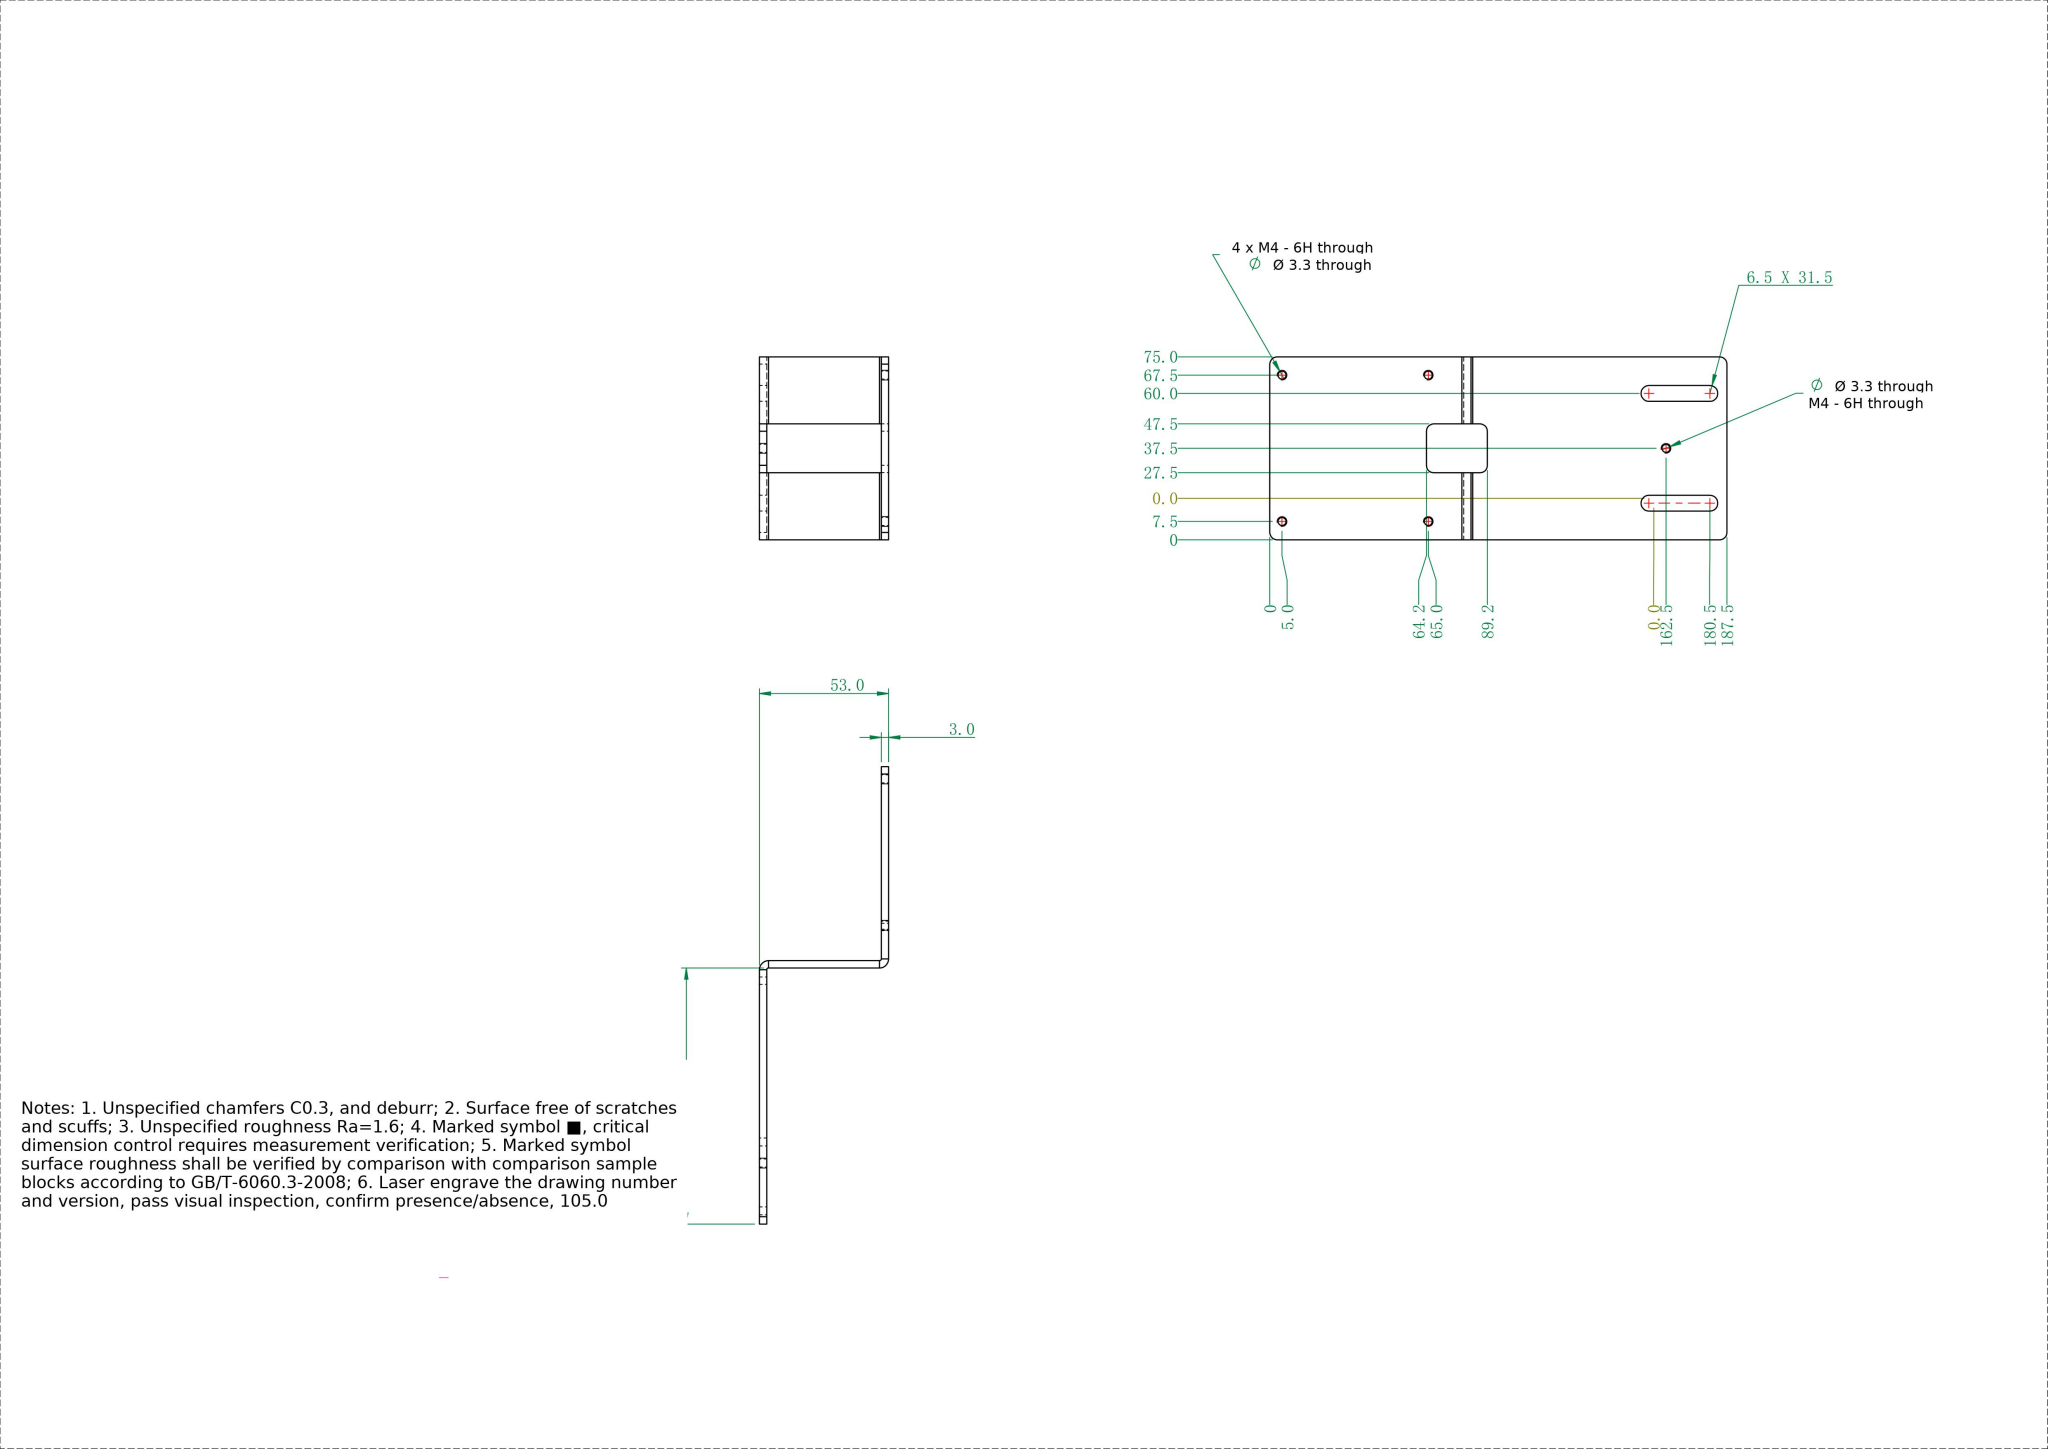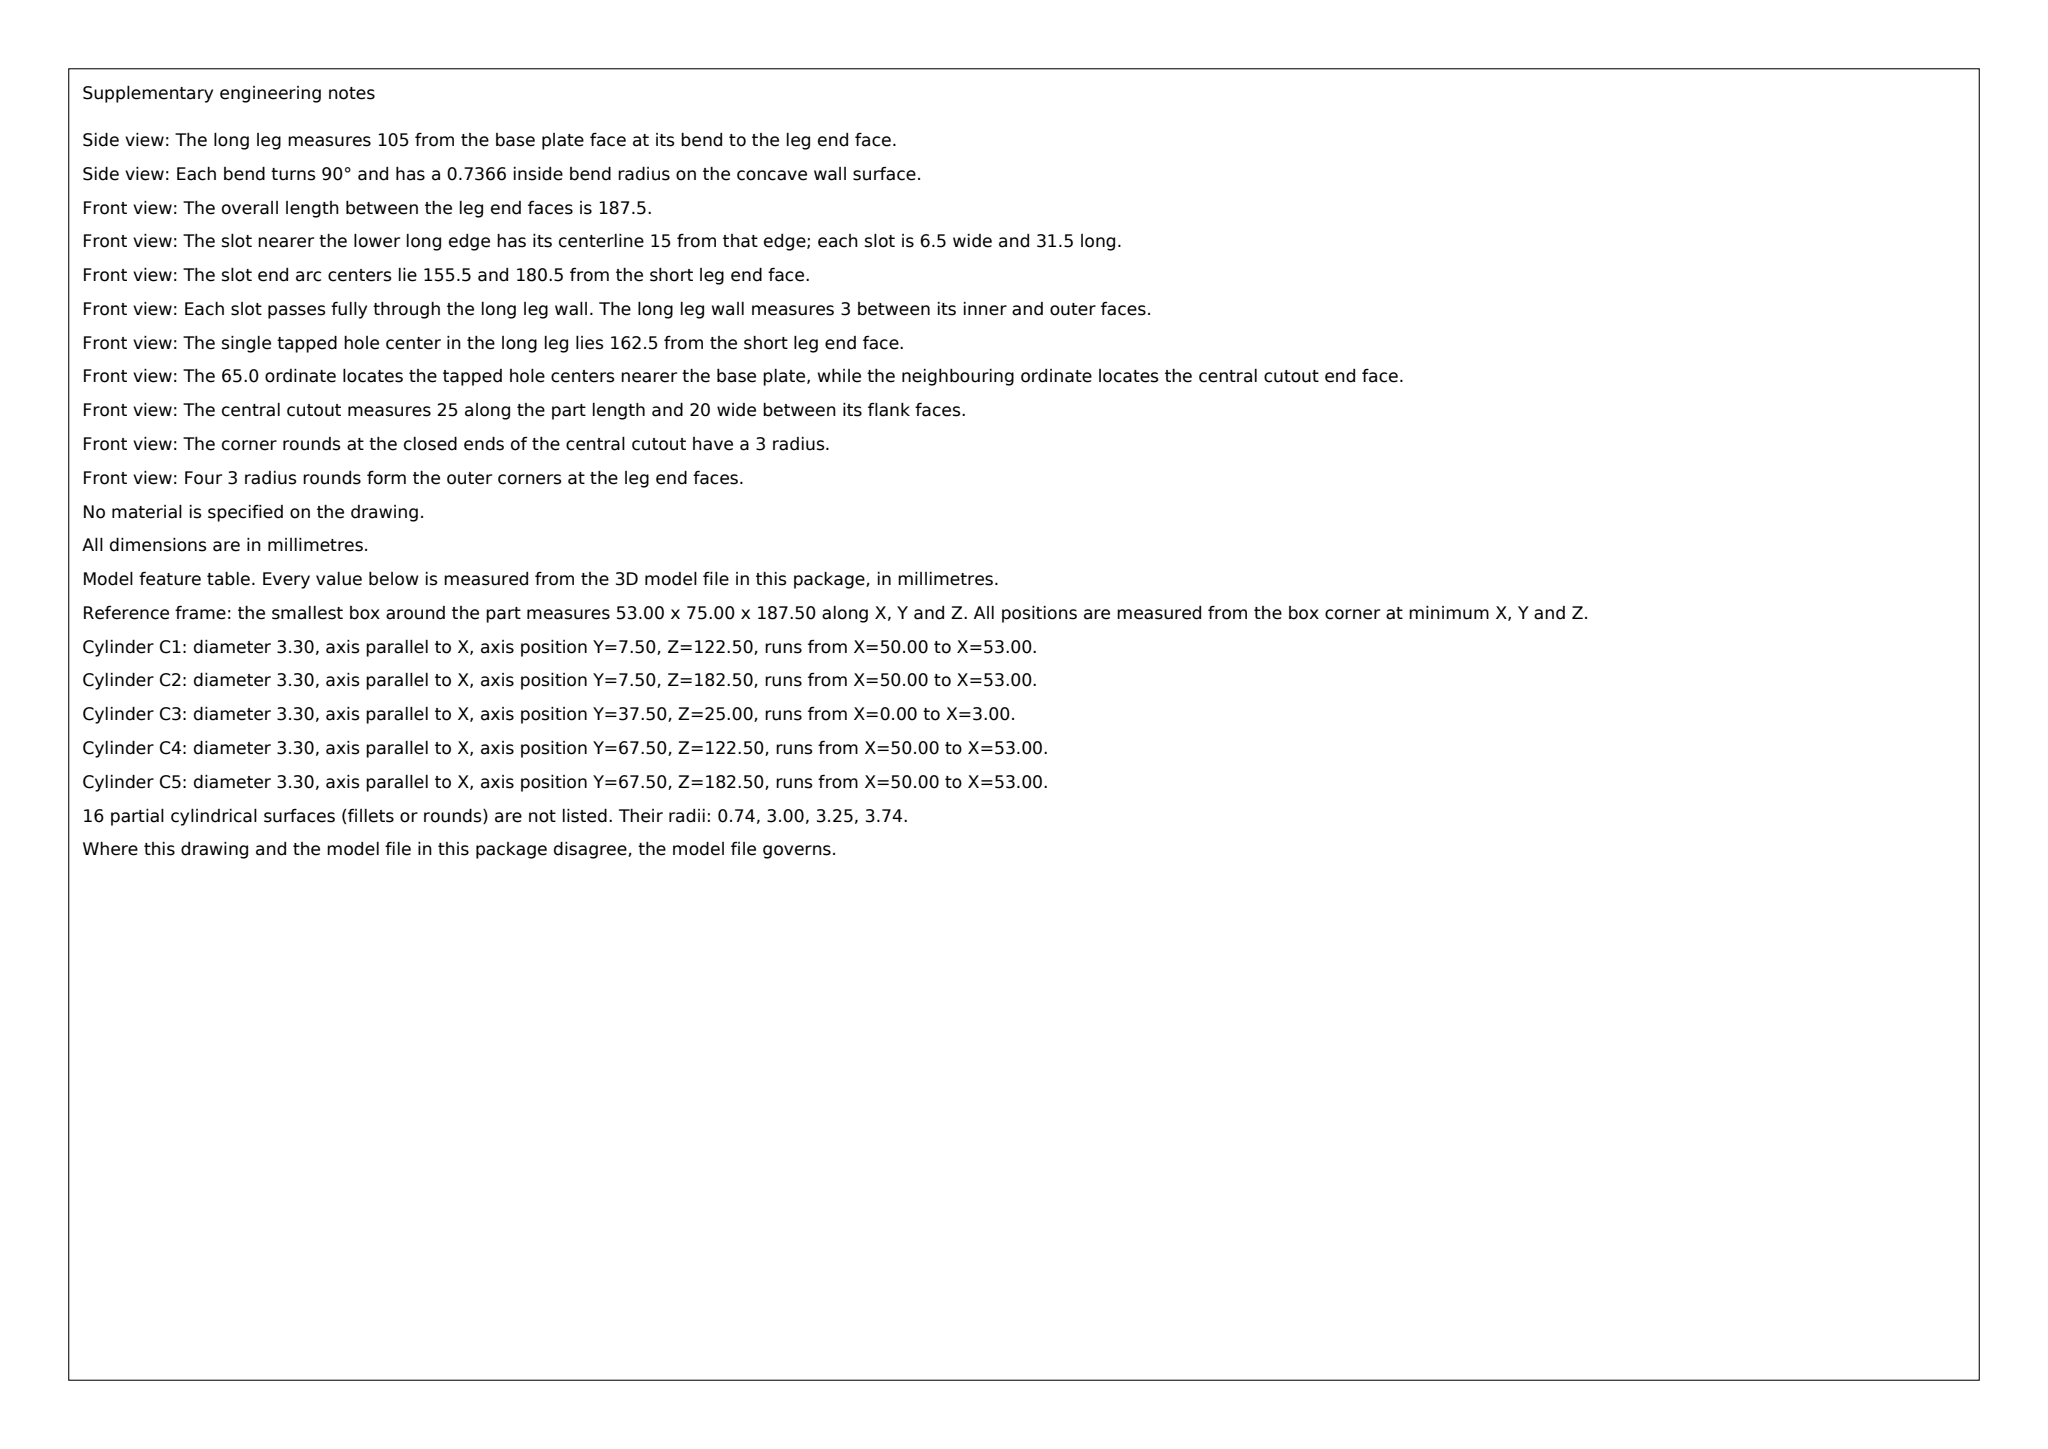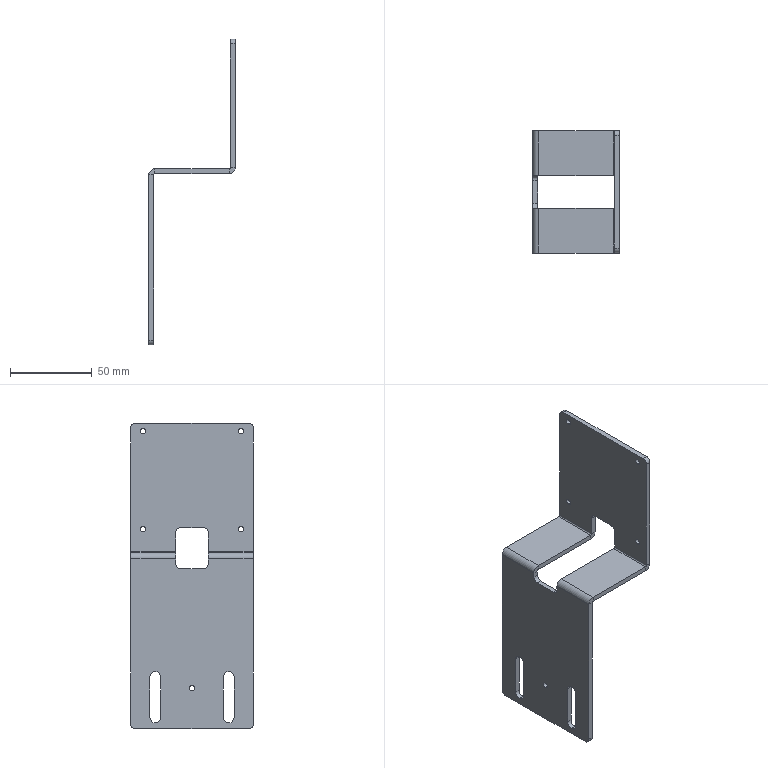Part | SolidWorks | mm | 1 solid | 68 faces | box 53 x 75 x 187.5 mm | volume 47318 mm3 | plane 36 | cylinder 32 | commonest cylinder face diameters 3.3 x10 6 x8 6.5 x6 7.473 x4 1.473 x4